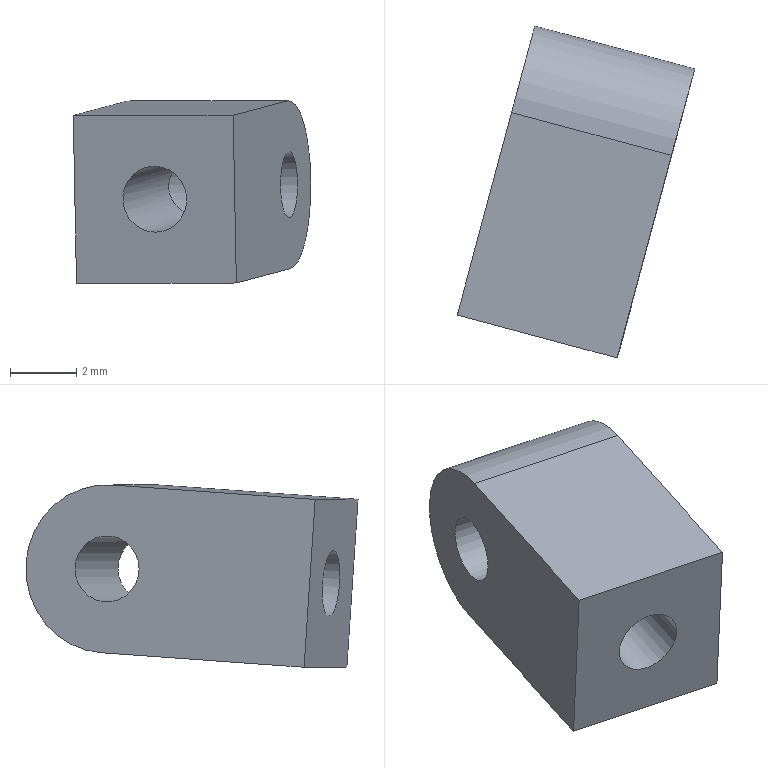Component | NX | BLOCK | 1 solid | 10 faces | box 7.18 x 10.03 x 5.52 mm | volume 179 mm3 | plane 5 | cylinder 3 | cone 2 | commonest cylinder face diameters 2 x2 5.08 x1
STEP:
#1=CARTESIAN_POINT('',(0.,0.,0.));
#2=DIRECTION('',(0.,0.,1.));
#3=DIRECTION('',(1.,0.,0.));
#4=AXIS2_PLACEMENT_3D('',#1,#2,#3);
#5=CARTESIAN_POINT('',(26.408,-132.214,153.506));
#6=VERTEX_POINT('',#5);
#7=CARTESIAN_POINT('',(28.048,-126.095,153.942));
#8=VERTEX_POINT('',#7);
#9=CARTESIAN_POINT('',(26.408,-132.214,153.506));
#10=DIRECTION('',(0.2582,0.9636,0.06876));
#11=VECTOR('',#10,1.);
#12=LINE('',#9,#11);
#13=CARTESIAN_POINT('',(21.579,-130.92,153.499));
#14=DIRECTION('',(0.01913,0.06606,-0.9976));
#15=DIRECTION('',(0.2582,0.9636,0.06876));
#16=AXIS2_PLACEMENT_3D('',#13,#14,#15);
#17=PLANE('',#16);
#18=CARTESIAN_POINT('',(0.,5.));
#19=DIRECTION('',(1.,0.));
#20=VECTOR('',#19,1.);
#21=LINE('',#18,#20);
#22=(GEOMETRIC_REPRESENTATION_CONTEXT(2)PARAMETRIC_REPRESENTATION_CONTEXT()REPRESENTATION_CONTEXT('',''));
#23=DEFINITIONAL_REPRESENTATION('',(#21),#22);
#24=PCURVE('',#17,#23);
#25=CARTESIAN_POINT('',(27.999,-126.263,156.476));
#26=DIRECTION('',(0.9659,-0.2589,0.001382));
#27=DIRECTION('',(0.2582,0.9636,0.06876));
#28=AXIS2_PLACEMENT_3D('',#25,#26,#27);
#29=PLANE('',#28);
#30=CARTESIAN_POINT('',(-6.35,-2.54));
#31=DIRECTION('',(1.,-0.));
#32=VECTOR('',#31,1.);
#33=LINE('',#30,#32);
#34=(GEOMETRIC_REPRESENTATION_CONTEXT(2)PARAMETRIC_REPRESENTATION_CONTEXT()REPRESENTATION_CONTEXT('',''));
#35=DEFINITIONAL_REPRESENTATION('',(#33),#34);
#36=PCURVE('',#29,#35);
#37=SURFACE_CURVE('',#12,(#24,#36),.PCURVE_S1.);
#38=EDGE_CURVE('',#6,#8,#37,.T.);
#39=ORIENTED_EDGE('',*,*,#38,.F.);
#40=CARTESIAN_POINT('',(21.579,-130.92,153.499));
#41=VERTEX_POINT('',#40);
#42=CARTESIAN_POINT('',(21.579,-130.92,153.499));
#43=DIRECTION('',(0.9659,-0.2589,0.001382));
#44=VECTOR('',#43,1.);
#45=LINE('',#42,#44);
#46=CARTESIAN_POINT('',(0.,0.));
#47=DIRECTION('',(-0.,1.));
#48=VECTOR('',#47,1.);
#49=LINE('',#46,#48);
#50=(GEOMETRIC_REPRESENTATION_CONTEXT(2)PARAMETRIC_REPRESENTATION_CONTEXT()REPRESENTATION_CONTEXT('',''));
#51=DEFINITIONAL_REPRESENTATION('',(#49),#50);
#52=PCURVE('',#17,#51);
#53=CARTESIAN_POINT('',(21.481,-131.255,158.567));
#54=DIRECTION('',(-0.2582,-0.9636,-0.06876));
#55=DIRECTION('',(0.01913,0.06606,-0.9976));
#56=AXIS2_PLACEMENT_3D('',#53,#54,#55);
#57=PLANE('',#56);
#58=CARTESIAN_POINT('',(5.08,0.));
#59=DIRECTION('',(-0.,1.));
#60=VECTOR('',#59,1.);
#61=LINE('',#58,#60);
#62=(GEOMETRIC_REPRESENTATION_CONTEXT(2)PARAMETRIC_REPRESENTATION_CONTEXT()REPRESENTATION_CONTEXT('',''));
#63=DEFINITIONAL_REPRESENTATION('',(#61),#62);
#64=PCURVE('',#57,#63);
#65=SURFACE_CURVE('',#45,(#52,#64),.PCURVE_S1.);
#66=EDGE_CURVE('',#41,#6,#65,.T.);
#67=ORIENTED_EDGE('',*,*,#66,.F.);
#68=CARTESIAN_POINT('',(23.218,-124.801,153.935));
#69=VERTEX_POINT('',#68);
#70=CARTESIAN_POINT('',(21.579,-130.92,153.499));
#71=DIRECTION('',(0.2582,0.9636,0.06876));
#72=VECTOR('',#71,1.);
#73=LINE('',#70,#72);
#74=CARTESIAN_POINT('',(0.,0.));
#75=DIRECTION('',(1.,0.));
#76=VECTOR('',#75,1.);
#77=LINE('',#74,#76);
#78=(GEOMETRIC_REPRESENTATION_CONTEXT(2)PARAMETRIC_REPRESENTATION_CONTEXT()REPRESENTATION_CONTEXT('',''));
#79=DEFINITIONAL_REPRESENTATION('',(#77),#78);
#80=PCURVE('',#17,#79);
#81=CARTESIAN_POINT('',(23.17,-124.969,156.469));
#82=DIRECTION('',(0.9659,-0.2589,0.001382));
#83=DIRECTION('',(0.2582,0.9636,0.06876));
#84=AXIS2_PLACEMENT_3D('',#81,#82,#83);
#85=PLANE('',#84);
#86=CARTESIAN_POINT('',(-6.35,-2.54));
#87=DIRECTION('',(1.,-0.));
#88=VECTOR('',#87,1.);
#89=LINE('',#86,#88);
#90=(GEOMETRIC_REPRESENTATION_CONTEXT(2)PARAMETRIC_REPRESENTATION_CONTEXT()REPRESENTATION_CONTEXT('',''));
#91=DEFINITIONAL_REPRESENTATION('',(#89),#90);
#92=PCURVE('',#85,#91);
#93=SURFACE_CURVE('',#73,(#80,#92),.PCURVE_S1.);
#94=EDGE_CURVE('',#41,#69,#93,.T.);
#95=ORIENTED_EDGE('',*,*,#94,.T.);
#96=CARTESIAN_POINT('',(23.218,-124.801,153.935));
#97=DIRECTION('',(0.9659,-0.2589,0.001382));
#98=VECTOR('',#97,1.);
#99=LINE('',#96,#98);
#100=CARTESIAN_POINT('',(6.35,-0.));
#101=DIRECTION('',(-0.,1.));
#102=VECTOR('',#101,1.);
#103=LINE('',#100,#102);
#104=(GEOMETRIC_REPRESENTATION_CONTEXT(2)PARAMETRIC_REPRESENTATION_CONTEXT()REPRESENTATION_CONTEXT('',''));
#105=DEFINITIONAL_REPRESENTATION('',(#103),#104);
#106=PCURVE('',#17,#105);
#107=CARTESIAN_POINT('',(23.17,-124.969,156.469));
#108=DIRECTION('',(0.9659,-0.2589,0.001382));
#109=DIRECTION('',(-0.01913,-0.06606,0.9976));
#110=AXIS2_PLACEMENT_3D('',#107,#108,#109);
#111=CYLINDRICAL_SURFACE('',#110,2.54);
#112=CARTESIAN_POINT('',(3.142,-0.));
#113=DIRECTION('',(-0.,1.));
#114=VECTOR('',#113,1.);
#115=LINE('',#112,#114);
#116=(GEOMETRIC_REPRESENTATION_CONTEXT(2)PARAMETRIC_REPRESENTATION_CONTEXT()REPRESENTATION_CONTEXT('',''));
#117=DEFINITIONAL_REPRESENTATION('',(#115),#116);
#118=PCURVE('',#111,#117);
#119=SURFACE_CURVE('',#99,(#106,#118),.PCURVE_S1.);
#120=EDGE_CURVE('',#69,#8,#119,.T.);
#121=ORIENTED_EDGE('',*,*,#120,.T.);
#122=EDGE_LOOP('',(#39,#67,#95,#121));
#123=FACE_BOUND('',#122,.T.);
#124=ADVANCED_FACE('',(#123),#17,.T.);
#125=CARTESIAN_POINT('',(27.951,-126.431,159.01));
#126=VERTEX_POINT('',#125);
#127=CARTESIAN_POINT('',(27.999,-126.263,156.476));
#128=DIRECTION('',(0.9659,-0.2589,0.001382));
#129=DIRECTION('',(0.2582,0.9636,0.06876));
#130=AXIS2_PLACEMENT_3D('',#127,#128,#129);
#131=CIRCLE('',#130,2.54);
#132=CARTESIAN_POINT('',(-1.571,5.));
#133=DIRECTION('',(1.,0.));
#134=VECTOR('',#133,1.);
#135=LINE('',#132,#134);
#136=(GEOMETRIC_REPRESENTATION_CONTEXT(2)PARAMETRIC_REPRESENTATION_CONTEXT()REPRESENTATION_CONTEXT('',''));
#137=DEFINITIONAL_REPRESENTATION('',(#135),#136);
#138=PCURVE('',#111,#137);
#139=CARTESIAN_POINT('',(0.,0.));
#140=DIRECTION('',(1.,0.));
#141=AXIS2_PLACEMENT_2D('',#139,#140);
#142=CIRCLE('',#141,2.54);
#143=(GEOMETRIC_REPRESENTATION_CONTEXT(2)PARAMETRIC_REPRESENTATION_CONTEXT()REPRESENTATION_CONTEXT('',''));
#144=DEFINITIONAL_REPRESENTATION('',(#142),#143);
#145=PCURVE('',#29,#144);
#146=SURFACE_CURVE('',#131,(#138,#145),.PCURVE_S1.);
#147=EDGE_CURVE('',#8,#126,#146,.T.);
#148=ORIENTED_EDGE('',*,*,#147,.F.);
#149=ORIENTED_EDGE('',*,*,#120,.F.);
#150=CARTESIAN_POINT('',(23.121,-125.136,159.003));
#151=VERTEX_POINT('',#150);
#152=CARTESIAN_POINT('',(23.17,-124.969,156.469));
#153=DIRECTION('',(0.9659,-0.2589,0.001382));
#154=DIRECTION('',(0.2582,0.9636,0.06876));
#155=AXIS2_PLACEMENT_3D('',#152,#153,#154);
#156=CIRCLE('',#155,2.54);
#157=CARTESIAN_POINT('',(-1.571,-0.));
#158=DIRECTION('',(1.,0.));
#159=VECTOR('',#158,1.);
#160=LINE('',#157,#159);
#161=(GEOMETRIC_REPRESENTATION_CONTEXT(2)PARAMETRIC_REPRESENTATION_CONTEXT()REPRESENTATION_CONTEXT('',''));
#162=DEFINITIONAL_REPRESENTATION('',(#160),#161);
#163=PCURVE('',#111,#162);
#164=CARTESIAN_POINT('',(0.,0.));
#165=DIRECTION('',(1.,0.));
#166=AXIS2_PLACEMENT_2D('',#164,#165);
#167=CIRCLE('',#166,2.54);
#168=(GEOMETRIC_REPRESENTATION_CONTEXT(2)PARAMETRIC_REPRESENTATION_CONTEXT()REPRESENTATION_CONTEXT('',''));
#169=DEFINITIONAL_REPRESENTATION('',(#167),#168);
#170=PCURVE('',#85,#169);
#171=SURFACE_CURVE('',#156,(#163,#170),.PCURVE_S1.);
#172=EDGE_CURVE('',#69,#151,#171,.T.);
#173=ORIENTED_EDGE('',*,*,#172,.T.);
#174=CARTESIAN_POINT('',(23.121,-125.136,159.003));
#175=DIRECTION('',(0.9659,-0.2589,0.001382));
#176=VECTOR('',#175,1.);
#177=LINE('',#174,#176);
#178=CARTESIAN_POINT('',(6.283,0.));
#179=DIRECTION('',(0.,1.));
#180=VECTOR('',#179,1.);
#181=LINE('',#178,#180);
#182=(GEOMETRIC_REPRESENTATION_CONTEXT(2)PARAMETRIC_REPRESENTATION_CONTEXT()REPRESENTATION_CONTEXT('',''));
#183=DEFINITIONAL_REPRESENTATION('',(#181),#182);
#184=PCURVE('',#111,#183);
#185=CARTESIAN_POINT('',(23.121,-125.136,159.003));
#186=DIRECTION('',(-0.01913,-0.06606,0.9976));
#187=DIRECTION('',(-0.2582,-0.9636,-0.06876));
#188=AXIS2_PLACEMENT_3D('',#185,#186,#187);
#189=PLANE('',#188);
#190=CARTESIAN_POINT('',(0.,0.));
#191=DIRECTION('',(0.,1.));
#192=VECTOR('',#191,1.);
#193=LINE('',#190,#192);
#194=(GEOMETRIC_REPRESENTATION_CONTEXT(2)PARAMETRIC_REPRESENTATION_CONTEXT()REPRESENTATION_CONTEXT('',''));
#195=DEFINITIONAL_REPRESENTATION('',(#193),#194);
#196=PCURVE('',#189,#195);
#197=SURFACE_CURVE('',#177,(#184,#196),.PCURVE_S1.);
#198=EDGE_CURVE('',#151,#126,#197,.T.);
#199=ORIENTED_EDGE('',*,*,#198,.T.);
#200=EDGE_LOOP('',(#148,#149,#173,#199));
#201=FACE_BOUND('',#200,.T.);
#202=ADVANCED_FACE('',(#201),#111,.T.);
#203=CARTESIAN_POINT('',(26.311,-132.55,158.574));
#204=VERTEX_POINT('',#203);
#205=CARTESIAN_POINT('',(27.951,-126.431,159.01));
#206=DIRECTION('',(-0.2582,-0.9636,-0.06876));
#207=VECTOR('',#206,1.);
#208=LINE('',#205,#207);
#209=CARTESIAN_POINT('',(-0.,5.));
#210=DIRECTION('',(1.,-0.));
#211=VECTOR('',#210,1.);
#212=LINE('',#209,#211);
#213=(GEOMETRIC_REPRESENTATION_CONTEXT(2)PARAMETRIC_REPRESENTATION_CONTEXT()REPRESENTATION_CONTEXT('',''));
#214=DEFINITIONAL_REPRESENTATION('',(#212),#213);
#215=PCURVE('',#189,#214);
#216=CARTESIAN_POINT('',(0.,2.54));
#217=DIRECTION('',(-1.,0.));
#218=VECTOR('',#217,1.);
#219=LINE('',#216,#218);
#220=(GEOMETRIC_REPRESENTATION_CONTEXT(2)PARAMETRIC_REPRESENTATION_CONTEXT()REPRESENTATION_CONTEXT('',''));
#221=DEFINITIONAL_REPRESENTATION('',(#219),#220);
#222=PCURVE('',#29,#221);
#223=SURFACE_CURVE('',#208,(#215,#222),.PCURVE_S1.);
#224=EDGE_CURVE('',#126,#204,#223,.T.);
#225=ORIENTED_EDGE('',*,*,#224,.F.);
#226=ORIENTED_EDGE('',*,*,#198,.F.);
#227=CARTESIAN_POINT('',(21.481,-131.255,158.567));
#228=VERTEX_POINT('',#227);
#229=CARTESIAN_POINT('',(23.121,-125.136,159.003));
#230=DIRECTION('',(-0.2582,-0.9636,-0.06876));
#231=VECTOR('',#230,1.);
#232=LINE('',#229,#231);
#233=CARTESIAN_POINT('',(0.,0.));
#234=DIRECTION('',(1.,-0.));
#235=VECTOR('',#234,1.);
#236=LINE('',#233,#235);
#237=(GEOMETRIC_REPRESENTATION_CONTEXT(2)PARAMETRIC_REPRESENTATION_CONTEXT()REPRESENTATION_CONTEXT('',''));
#238=DEFINITIONAL_REPRESENTATION('',(#236),#237);
#239=PCURVE('',#189,#238);
#240=CARTESIAN_POINT('',(0.,2.54));
#241=DIRECTION('',(-1.,0.));
#242=VECTOR('',#241,1.);
#243=LINE('',#240,#242);
#244=(GEOMETRIC_REPRESENTATION_CONTEXT(2)PARAMETRIC_REPRESENTATION_CONTEXT()REPRESENTATION_CONTEXT('',''));
#245=DEFINITIONAL_REPRESENTATION('',(#243),#244);
#246=PCURVE('',#85,#245);
#247=SURFACE_CURVE('',#232,(#239,#246),.PCURVE_S1.);
#248=EDGE_CURVE('',#151,#228,#247,.T.);
#249=ORIENTED_EDGE('',*,*,#248,.T.);
#250=CARTESIAN_POINT('',(21.481,-131.255,158.567));
#251=DIRECTION('',(0.9659,-0.2589,0.001382));
#252=VECTOR('',#251,1.);
#253=LINE('',#250,#252);
#254=CARTESIAN_POINT('',(6.35,-0.));
#255=DIRECTION('',(0.,1.));
#256=VECTOR('',#255,1.);
#257=LINE('',#254,#256);
#258=(GEOMETRIC_REPRESENTATION_CONTEXT(2)PARAMETRIC_REPRESENTATION_CONTEXT()REPRESENTATION_CONTEXT('',''));
#259=DEFINITIONAL_REPRESENTATION('',(#257),#258);
#260=PCURVE('',#189,#259);
#261=CARTESIAN_POINT('',(0.,0.));
#262=DIRECTION('',(-0.,1.));
#263=VECTOR('',#262,1.);
#264=LINE('',#261,#263);
#265=(GEOMETRIC_REPRESENTATION_CONTEXT(2)PARAMETRIC_REPRESENTATION_CONTEXT()REPRESENTATION_CONTEXT('',''));
#266=DEFINITIONAL_REPRESENTATION('',(#264),#265);
#267=PCURVE('',#57,#266);
#268=SURFACE_CURVE('',#253,(#260,#267),.PCURVE_S1.);
#269=EDGE_CURVE('',#228,#204,#268,.T.);
#270=ORIENTED_EDGE('',*,*,#269,.T.);
#271=EDGE_LOOP('',(#225,#226,#249,#270));
#272=FACE_BOUND('',#271,.T.);
#273=ADVANCED_FACE('',(#272),#189,.T.);
#274=CARTESIAN_POINT('',(23.926,-131.801,157.034));
#275=VERTEX_POINT('',#274);
#276=CARTESIAN_POINT('',(23.945,-131.735,156.036));
#277=DIRECTION('',(0.2582,0.9636,0.06876));
#278=DIRECTION('',(-0.01913,-0.06606,0.9976));
#279=AXIS2_PLACEMENT_3D('',#276,#277,#278);
#280=CIRCLE('',#279,1.);
#281=CARTESIAN_POINT('',(1.54,2.5));
#282=CARTESIAN_POINT('',(1.54,4.232));
#283=CARTESIAN_POINT('',(3.04,3.366));
#284=CARTESIAN_POINT('',(4.54,2.5));
#285=CARTESIAN_POINT('',(3.04,1.634));
#286=CARTESIAN_POINT('',(1.54,0.7679));
#287=CARTESIAN_POINT('',(1.54,2.5));
#288=(BOUNDED_CURVE()B_SPLINE_CURVE(2,(#281,#282,#283,#284,#285,#286,#287),.UNSPECIFIED.,.T.,.F.)B_SPLINE_CURVE_WITH_KNOTS((1,2,2,2,2,1),(-2.094,0.,2.094,4.189,6.283,8.378),.UNSPECIFIED.)CURVE()GEOMETRIC_REPRESENTATION_ITEM()RATIONAL_B_SPLINE_CURVE((1.,0.5,1.,0.5,1.,0.5,1.))REPRESENTATION_ITEM(''));
#289=(GEOMETRIC_REPRESENTATION_CONTEXT(2)PARAMETRIC_REPRESENTATION_CONTEXT()REPRESENTATION_CONTEXT('',''));
#290=DEFINITIONAL_REPRESENTATION('',(#288),#289);
#291=PCURVE('',#57,#290);
#292=CARTESIAN_POINT('',(23.945,-131.735,156.036));
#293=DIRECTION('',(0.2582,0.9636,0.06876));
#294=DIRECTION('',(-0.01913,-0.06606,0.9976));
#295=AXIS2_PLACEMENT_3D('',#292,#293,#294);
#296=CYLINDRICAL_SURFACE('',#295,1.);
#297=CARTESIAN_POINT('',(0.,0.));
#298=DIRECTION('',(1.,0.));
#299=VECTOR('',#298,1.);
#300=LINE('',#297,#299);
#301=(GEOMETRIC_REPRESENTATION_CONTEXT(2)PARAMETRIC_REPRESENTATION_CONTEXT()REPRESENTATION_CONTEXT('',''));
#302=DEFINITIONAL_REPRESENTATION('',(#300),#301);
#303=PCURVE('',#296,#302);
#304=SURFACE_CURVE('',#280,(#291,#303),.PCURVE_S1.);
#305=EDGE_CURVE('',#275,#275,#304,.T.);
#306=ORIENTED_EDGE('',*,*,#305,.T.);
#307=EDGE_LOOP('',(#306));
#308=FACE_BOUND('',#307,.T.);
#309=CARTESIAN_POINT('',(26.311,-132.55,158.574));
#310=DIRECTION('',(0.01913,0.06606,-0.9976));
#311=VECTOR('',#310,1.);
#312=LINE('',#309,#311);
#313=CARTESIAN_POINT('',(-0.,5.));
#314=DIRECTION('',(1.,-0.));
#315=VECTOR('',#314,1.);
#316=LINE('',#313,#315);
#317=(GEOMETRIC_REPRESENTATION_CONTEXT(2)PARAMETRIC_REPRESENTATION_CONTEXT()REPRESENTATION_CONTEXT('',''));
#318=DEFINITIONAL_REPRESENTATION('',(#316),#317);
#319=PCURVE('',#57,#318);
#320=CARTESIAN_POINT('',(-6.35,2.54));
#321=DIRECTION('',(0.,-1.));
#322=VECTOR('',#321,1.);
#323=LINE('',#320,#322);
#324=(GEOMETRIC_REPRESENTATION_CONTEXT(2)PARAMETRIC_REPRESENTATION_CONTEXT()REPRESENTATION_CONTEXT('',''));
#325=DEFINITIONAL_REPRESENTATION('',(#323),#324);
#326=PCURVE('',#29,#325);
#327=SURFACE_CURVE('',#312,(#319,#326),.PCURVE_S1.);
#328=EDGE_CURVE('',#204,#6,#327,.T.);
#329=ORIENTED_EDGE('',*,*,#328,.F.);
#330=ORIENTED_EDGE('',*,*,#269,.F.);
#331=CARTESIAN_POINT('',(21.481,-131.255,158.567));
#332=DIRECTION('',(0.01913,0.06606,-0.9976));
#333=VECTOR('',#332,1.);
#334=LINE('',#331,#333);
#335=CARTESIAN_POINT('',(0.,0.));
#336=DIRECTION('',(1.,-0.));
#337=VECTOR('',#336,1.);
#338=LINE('',#335,#337);
#339=(GEOMETRIC_REPRESENTATION_CONTEXT(2)PARAMETRIC_REPRESENTATION_CONTEXT()REPRESENTATION_CONTEXT('',''));
#340=DEFINITIONAL_REPRESENTATION('',(#338),#339);
#341=PCURVE('',#57,#340);
#342=CARTESIAN_POINT('',(-6.35,2.54));
#343=DIRECTION('',(0.,-1.));
#344=VECTOR('',#343,1.);
#345=LINE('',#342,#344);
#346=(GEOMETRIC_REPRESENTATION_CONTEXT(2)PARAMETRIC_REPRESENTATION_CONTEXT()REPRESENTATION_CONTEXT('',''));
#347=DEFINITIONAL_REPRESENTATION('',(#345),#346);
#348=PCURVE('',#85,#347);
#349=SURFACE_CURVE('',#334,(#341,#348),.PCURVE_S1.);
#350=EDGE_CURVE('',#228,#41,#349,.T.);
#351=ORIENTED_EDGE('',*,*,#350,.T.);
#352=ORIENTED_EDGE('',*,*,#66,.T.);
#353=EDGE_LOOP('',(#329,#330,#351,#352));
#354=FACE_BOUND('',#353,.T.);
#355=ADVANCED_FACE('',(#308,#354),#57,.T.);
#356=CARTESIAN_POINT('',(23.429,-124.003,156.469));
#357=VERTEX_POINT('',#356);
#358=CARTESIAN_POINT('',(23.17,-124.969,156.469));
#359=DIRECTION('',(0.9659,-0.2589,0.001382));
#360=DIRECTION('',(0.2589,0.9659,0.00000007));
#361=AXIS2_PLACEMENT_3D('',#358,#359,#360);
#362=CIRCLE('',#361,1.);
#363=CARTESIAN_POINT('',(23.17,-124.969,156.469));
#364=DIRECTION('',(0.9659,-0.2589,0.001382));
#365=DIRECTION('',(-0.01913,-0.06606,0.9976));
#366=AXIS2_PLACEMENT_3D('',#363,#364,#365);
#367=CYLINDRICAL_SURFACE('',#366,1.);
#368=CARTESIAN_POINT('',(4.644,0.));
#369=DIRECTION('',(1.,0.));
#370=VECTOR('',#369,1.);
#371=LINE('',#368,#370);
#372=(GEOMETRIC_REPRESENTATION_CONTEXT(2)PARAMETRIC_REPRESENTATION_CONTEXT()REPRESENTATION_CONTEXT('',''));
#373=DEFINITIONAL_REPRESENTATION('',(#371),#372);
#374=PCURVE('',#367,#373);
#375=CARTESIAN_POINT('',(0.,-0.));
#376=DIRECTION('',(0.9976,-0.06876));
#377=AXIS2_PLACEMENT_2D('',#375,#376);
#378=CIRCLE('',#377,1.);
#379=(GEOMETRIC_REPRESENTATION_CONTEXT(2)PARAMETRIC_REPRESENTATION_CONTEXT()REPRESENTATION_CONTEXT('',''));
#380=DEFINITIONAL_REPRESENTATION('',(#378),#379);
#381=PCURVE('',#85,#380);
#382=SURFACE_CURVE('',#362,(#374,#381),.PCURVE_S1.);
#383=EDGE_CURVE('',#357,#357,#382,.T.);
#384=ORIENTED_EDGE('',*,*,#383,.T.);
#385=CARTESIAN_POINT('',(28.258,-125.297,156.476));
#386=VERTEX_POINT('',#385);
#387=CARTESIAN_POINT('',(23.429,-124.003,156.469));
#388=CARTESIAN_POINT('',(28.258,-125.297,156.476));
#389=B_SPLINE_CURVE_WITH_KNOTS('',1,(#387,#388),.UNSPECIFIED.,.F.,.F.,(2,2),(0.,5.),.PIECEWISE_BEZIER_KNOTS.);
#390=CARTESIAN_POINT('',(10.927,0.));
#391=DIRECTION('',(0.,1.));
#392=VECTOR('',#391,1.);
#393=LINE('',#390,#392);
#394=(GEOMETRIC_REPRESENTATION_CONTEXT(2)PARAMETRIC_REPRESENTATION_CONTEXT()REPRESENTATION_CONTEXT('',''));
#395=DEFINITIONAL_REPRESENTATION('',(#393),#394);
#396=PCURVE('',#367,#395);
#397=CARTESIAN_POINT('',(4.644,0.));
#398=DIRECTION('',(0.,1.));
#399=VECTOR('',#398,1.);
#400=LINE('',#397,#399);
#401=(GEOMETRIC_REPRESENTATION_CONTEXT(2)PARAMETRIC_REPRESENTATION_CONTEXT()REPRESENTATION_CONTEXT('',''));
#402=DEFINITIONAL_REPRESENTATION('',(#400),#401);
#403=PCURVE('',#367,#402);
#404=SEAM_CURVE('',#389,(#396,#403),.PCURVE_S1.);
#405=EDGE_CURVE('',#357,#386,#404,.T.);
#406=ORIENTED_EDGE('',*,*,#405,.T.);
#407=CARTESIAN_POINT('',(27.999,-126.263,156.476));
#408=DIRECTION('',(0.9659,-0.2589,0.001382));
#409=DIRECTION('',(0.2589,0.9659,0.00000007));
#410=AXIS2_PLACEMENT_3D('',#407,#408,#409);
#411=CIRCLE('',#410,1.);
#412=CARTESIAN_POINT('',(4.644,5.));
#413=DIRECTION('',(1.,0.));
#414=VECTOR('',#413,1.);
#415=LINE('',#412,#414);
#416=(GEOMETRIC_REPRESENTATION_CONTEXT(2)PARAMETRIC_REPRESENTATION_CONTEXT()REPRESENTATION_CONTEXT('',''));
#417=DEFINITIONAL_REPRESENTATION('',(#415),#416);
#418=PCURVE('',#367,#417);
#419=CARTESIAN_POINT('',(0.,-0.));
#420=DIRECTION('',(0.9976,-0.06876));
#421=AXIS2_PLACEMENT_2D('',#419,#420);
#422=CIRCLE('',#421,1.);
#423=(GEOMETRIC_REPRESENTATION_CONTEXT(2)PARAMETRIC_REPRESENTATION_CONTEXT()REPRESENTATION_CONTEXT('',''));
#424=DEFINITIONAL_REPRESENTATION('',(#422),#423);
#425=PCURVE('',#29,#424);
#426=SURFACE_CURVE('',#411,(#418,#425),.PCURVE_S1.);
#427=EDGE_CURVE('',#386,#386,#426,.T.);
#428=ORIENTED_EDGE('',*,*,#427,.F.);
#429=ORIENTED_EDGE('',*,*,#405,.F.);
#430=EDGE_LOOP('',(#384,#406,#428,#429));
#431=FACE_BOUND('',#430,.F.);
#432=CARTESIAN_POINT('',(25.138,-125.924,157.383));
#433=VERTEX_POINT('',#432);
#434=CARTESIAN_POINT('',(25.174,-125.801,155.514));
#435=VERTEX_POINT('',#434);
#436=CARTESIAN_POINT('',(25.584,-125.616,156.473));
#437=DIRECTION('',(0.5004,-0.8645,-0.04764));
#438=DIRECTION('',(0.8656,0.4983,0.0496));
#439=AXIS2_PLACEMENT_3D('',#436,#437,#438);
#440=ELLIPSE('',#439,1.414,1.);
#441=CARTESIAN_POINT('',(6.641,2.15));
#442=CARTESIAN_POINT('',(6.678,2.116));
#443=CARTESIAN_POINT('',(6.751,2.048));
#444=CARTESIAN_POINT('',(6.861,1.952));
#445=CARTESIAN_POINT('',(6.972,1.863));
#446=CARTESIAN_POINT('',(7.082,1.782));
#447=CARTESIAN_POINT('',(7.192,1.709));
#448=CARTESIAN_POINT('',(7.303,1.647));
#449=CARTESIAN_POINT('',(7.413,1.594));
#450=CARTESIAN_POINT('',(7.523,1.552));
#451=CARTESIAN_POINT('',(7.633,1.522));
#452=CARTESIAN_POINT('',(7.744,1.504));
#453=CARTESIAN_POINT('',(7.854,1.498));
#454=CARTESIAN_POINT('',(7.964,1.504));
#455=CARTESIAN_POINT('',(8.075,1.522));
#456=CARTESIAN_POINT('',(8.185,1.552));
#457=CARTESIAN_POINT('',(8.295,1.594));
#458=CARTESIAN_POINT('',(8.405,1.647));
#459=CARTESIAN_POINT('',(8.516,1.709));
#460=CARTESIAN_POINT('',(8.626,1.782));
#461=CARTESIAN_POINT('',(8.736,1.863));
#462=CARTESIAN_POINT('',(8.847,1.952));
#463=CARTESIAN_POINT('',(8.957,2.048));
#464=CARTESIAN_POINT('',(9.03,2.116));
#465=CARTESIAN_POINT('',(9.067,2.15));
#466=B_SPLINE_CURVE_WITH_KNOTS('',3,(#441,#442,#443,#444,#445,#446,#447,#448,#449,#450,#451,#452,#453,#454,#455,#456,#457,#458,#459,#460,#461,#462,#463,#464,#465),.UNSPECIFIED.,.F.,.F.,(4,1,1,1,1,1,1,1,1,1,1,1,1,1,1,1,1,1,1,1,1,1,4),(1.928,2.039,2.149,2.259,2.37,2.48,2.59,2.7,2.811,2.921,3.031,3.142,3.252,3.362,3.472,3.583,3.693,3.803,3.914,4.024,4.134,4.245,4.355),.QUASI_UNIFORM_KNOTS.);
#467=(GEOMETRIC_REPRESENTATION_CONTEXT(2)PARAMETRIC_REPRESENTATION_CONTEXT()REPRESENTATION_CONTEXT('',''));
#468=DEFINITIONAL_REPRESENTATION('',(#466),#467);
#469=PCURVE('',#367,#468);
#470=CARTESIAN_POINT('',(5.926,6.));
#471=CARTESIAN_POINT('',(5.889,5.966));
#472=CARTESIAN_POINT('',(5.815,5.898));
#473=CARTESIAN_POINT('',(5.705,5.802));
#474=CARTESIAN_POINT('',(5.595,5.713));
#475=CARTESIAN_POINT('',(5.484,5.632));
#476=CARTESIAN_POINT('',(5.374,5.559));
#477=CARTESIAN_POINT('',(5.264,5.497));
#478=CARTESIAN_POINT('',(5.154,5.444));
#479=CARTESIAN_POINT('',(5.043,5.402));
#480=CARTESIAN_POINT('',(4.933,5.372));
#481=CARTESIAN_POINT('',(4.823,5.354));
#482=CARTESIAN_POINT('',(4.712,5.348));
#483=CARTESIAN_POINT('',(4.602,5.354));
#484=CARTESIAN_POINT('',(4.492,5.372));
#485=CARTESIAN_POINT('',(4.382,5.402));
#486=CARTESIAN_POINT('',(4.271,5.444));
#487=CARTESIAN_POINT('',(4.161,5.497));
#488=CARTESIAN_POINT('',(4.051,5.559));
#489=CARTESIAN_POINT('',(3.94,5.632));
#490=CARTESIAN_POINT('',(3.83,5.713));
#491=CARTESIAN_POINT('',(3.72,5.802));
#492=CARTESIAN_POINT('',(3.609,5.898));
#493=CARTESIAN_POINT('',(3.536,5.966));
#494=CARTESIAN_POINT('',(3.499,6.));
#495=B_SPLINE_CURVE_WITH_KNOTS('',3,(#470,#471,#472,#473,#474,#475,#476,#477,#478,#479,#480,#481,#482,#483,#484,#485,#486,#487,#488,#489,#490,#491,#492,#493,#494),.UNSPECIFIED.,.F.,.F.,(4,1,1,1,1,1,1,1,1,1,1,1,1,1,1,1,1,1,1,1,1,1,4),(1.928,2.039,2.149,2.259,2.37,2.48,2.59,2.7,2.811,2.921,3.031,3.142,3.252,3.362,3.472,3.583,3.693,3.803,3.914,4.024,4.134,4.245,4.355),.QUASI_UNIFORM_KNOTS.);
#496=(GEOMETRIC_REPRESENTATION_CONTEXT(2)PARAMETRIC_REPRESENTATION_CONTEXT()REPRESENTATION_CONTEXT('',''));
#497=DEFINITIONAL_REPRESENTATION('',(#495),#496);
#498=PCURVE('',#296,#497);
#499=SURFACE_CURVE('',#440,(#469,#498),.PCURVE_S1.);
#500=EDGE_CURVE('',#433,#435,#499,.T.);
#501=ORIENTED_EDGE('',*,*,#500,.F.);
#502=CARTESIAN_POINT('',(25.814,-126.106,157.384));
#503=VERTEX_POINT('',#502);
#504=CARTESIAN_POINT('',(25.814,-126.106,157.384));
#505=CARTESIAN_POINT('',(25.716,-126.061,157.392));
#506=CARTESIAN_POINT('',(25.614,-126.022,157.396));
#507=CARTESIAN_POINT('',(25.509,-125.993,157.396));
#508=CARTESIAN_POINT('',(25.388,-125.958,157.397));
#509=CARTESIAN_POINT('',(25.263,-125.936,157.392));
#510=CARTESIAN_POINT('',(25.138,-125.924,157.383));
#511=B_SPLINE_CURVE_WITH_KNOTS('',3,(#504,#505,#506,#507,#508,#509,#510),.UNSPECIFIED.,.F.,.F.,(4,3,4),(0.,0.4619,1.),.UNSPECIFIED.);
#512=CARTESIAN_POINT('',(6.641,2.85));
#513=CARTESIAN_POINT('',(6.639,2.84));
#514=CARTESIAN_POINT('',(6.635,2.818));
#515=CARTESIAN_POINT('',(6.63,2.787));
#516=CARTESIAN_POINT('',(6.625,2.755));
#517=CARTESIAN_POINT('',(6.621,2.723));
#518=CARTESIAN_POINT('',(6.618,2.692));
#519=CARTESIAN_POINT('',(6.615,2.66));
#520=CARTESIAN_POINT('',(6.612,2.628));
#521=CARTESIAN_POINT('',(6.61,2.596));
#522=CARTESIAN_POINT('',(6.609,2.564));
#523=CARTESIAN_POINT('',(6.608,2.532));
#524=CARTESIAN_POINT('',(6.607,2.5));
#525=CARTESIAN_POINT('',(6.608,2.468));
#526=CARTESIAN_POINT('',(6.609,2.436));
#527=CARTESIAN_POINT('',(6.61,2.404));
#528=CARTESIAN_POINT('',(6.612,2.372));
#529=CARTESIAN_POINT('',(6.615,2.34));
#530=CARTESIAN_POINT('',(6.618,2.308));
#531=CARTESIAN_POINT('',(6.621,2.276));
#532=CARTESIAN_POINT('',(6.625,2.245));
#533=CARTESIAN_POINT('',(6.63,2.213));
#534=CARTESIAN_POINT('',(6.635,2.181));
#535=CARTESIAN_POINT('',(6.639,2.16));
#536=CARTESIAN_POINT('',(6.641,2.15));
#537=B_SPLINE_CURVE_WITH_KNOTS('',3,(#512,#513,#514,#515,#516,#517,#518,#519,#520,#521,#522,#523,#524,#525,#526,#527,#528,#529,#530,#531,#532,#533,#534,#535,#536),.UNSPECIFIED.,.F.,.F.,(4,1,1,1,1,1,1,1,1,1,1,1,1,1,1,1,1,1,1,1,1,1,4),(0.,0.04545,0.09091,0.1364,0.1818,0.2273,0.2727,0.3182,0.3636,0.4091,0.4545,0.5,0.5455,0.5909,0.6364,0.6818,0.7273,0.7727,0.8182,0.8636,0.9091,0.9545,1.),.QUASI_UNIFORM_KNOTS.);
#538=(GEOMETRIC_REPRESENTATION_CONTEXT(2)PARAMETRIC_REPRESENTATION_CONTEXT()REPRESENTATION_CONTEXT('',''));
#539=DEFINITIONAL_REPRESENTATION('',(#537),#538);
#540=PCURVE('',#367,#539);
#541=CARTESIAN_POINT('',(25.494,-125.953,156.449));
#542=DIRECTION('',(-0.2582,-0.9636,-0.06876));
#543=DIRECTION('',(0.01913,0.06606,-0.9976));
#544=AXIS2_PLACEMENT_3D('',#541,#542,#543);
#545=CONICAL_SURFACE('',#544,1.,1.03);
#546=CARTESIAN_POINT('',(2.784,-0.));
#547=CARTESIAN_POINT('',(2.794,-0.001823));
#548=CARTESIAN_POINT('',(2.814,-0.005328));
#549=CARTESIAN_POINT('',(2.845,-0.01015));
#550=CARTESIAN_POINT('',(2.877,-0.01451));
#551=CARTESIAN_POINT('',(2.909,-0.01841));
#552=CARTESIAN_POINT('',(2.942,-0.02182));
#553=CARTESIAN_POINT('',(2.974,-0.02473));
#554=CARTESIAN_POINT('',(3.008,-0.02712));
#555=CARTESIAN_POINT('',(3.041,-0.029));
#556=CARTESIAN_POINT('',(3.074,-0.03035));
#557=CARTESIAN_POINT('',(3.108,-0.03115));
#558=CARTESIAN_POINT('',(3.142,-0.03141));
#559=CARTESIAN_POINT('',(3.176,-0.03113));
#560=CARTESIAN_POINT('',(3.209,-0.03031));
#561=CARTESIAN_POINT('',(3.243,-0.02896));
#562=CARTESIAN_POINT('',(3.276,-0.02708));
#563=CARTESIAN_POINT('',(3.309,-0.02468));
#564=CARTESIAN_POINT('',(3.342,-0.02177));
#565=CARTESIAN_POINT('',(3.374,-0.01837));
#566=CARTESIAN_POINT('',(3.406,-0.01448));
#567=CARTESIAN_POINT('',(3.438,-0.01012));
#568=CARTESIAN_POINT('',(3.469,-0.005314));
#569=CARTESIAN_POINT('',(3.489,-0.001818));
#570=CARTESIAN_POINT('',(3.499,-0.));
#571=B_SPLINE_CURVE_WITH_KNOTS('',3,(#546,#547,#548,#549,#550,#551,#552,#553,#554,#555,#556,#557,#558,#559,#560,#561,#562,#563,#564,#565,#566,#567,#568,#569,#570),.UNSPECIFIED.,.F.,.F.,(4,1,1,1,1,1,1,1,1,1,1,1,1,1,1,1,1,1,1,1,1,1,4),(0.,0.04545,0.09091,0.1364,0.1818,0.2273,0.2727,0.3182,0.3636,0.4091,0.4545,0.5,0.5455,0.5909,0.6364,0.6818,0.7273,0.7727,0.8182,0.8636,0.9091,0.9545,1.),.QUASI_UNIFORM_KNOTS.);
#572=(GEOMETRIC_REPRESENTATION_CONTEXT(2)PARAMETRIC_REPRESENTATION_CONTEXT()REPRESENTATION_CONTEXT('',''));
#573=DEFINITIONAL_REPRESENTATION('',(#571),#572);
#574=PCURVE('',#545,#573);
#575=SURFACE_CURVE('',#511,(#540,#574),.PCURVE_S1.);
#576=EDGE_CURVE('',#503,#433,#575,.T.);
#577=ORIENTED_EDGE('',*,*,#576,.F.);
#578=CARTESIAN_POINT('',(25.85,-125.982,155.515));
#579=VERTEX_POINT('',#578);
#580=CARTESIAN_POINT('',(25.584,-125.616,156.473));
#581=DIRECTION('',(-0.8656,-0.4983,-0.0496));
#582=DIRECTION('',(0.5004,-0.8645,-0.04764));
#583=AXIS2_PLACEMENT_3D('',#580,#581,#582);
#584=ELLIPSE('',#583,1.414,1.);
#585=CARTESIAN_POINT('',(9.067,2.85));
#586=CARTESIAN_POINT('',(9.03,2.884));
#587=CARTESIAN_POINT('',(8.957,2.952));
#588=CARTESIAN_POINT('',(8.847,3.048));
#589=CARTESIAN_POINT('',(8.736,3.137));
#590=CARTESIAN_POINT('',(8.626,3.218));
#591=CARTESIAN_POINT('',(8.516,3.291));
#592=CARTESIAN_POINT('',(8.405,3.353));
#593=CARTESIAN_POINT('',(8.295,3.406));
#594=CARTESIAN_POINT('',(8.185,3.448));
#595=CARTESIAN_POINT('',(8.075,3.478));
#596=CARTESIAN_POINT('',(7.964,3.496));
#597=CARTESIAN_POINT('',(7.854,3.502));
#598=CARTESIAN_POINT('',(7.744,3.496));
#599=CARTESIAN_POINT('',(7.633,3.478));
#600=CARTESIAN_POINT('',(7.523,3.448));
#601=CARTESIAN_POINT('',(7.413,3.406));
#602=CARTESIAN_POINT('',(7.303,3.353));
#603=CARTESIAN_POINT('',(7.192,3.291));
#604=CARTESIAN_POINT('',(7.082,3.218));
#605=CARTESIAN_POINT('',(6.972,3.137));
#606=CARTESIAN_POINT('',(6.861,3.048));
#607=CARTESIAN_POINT('',(6.751,2.952));
#608=CARTESIAN_POINT('',(6.678,2.884));
#609=CARTESIAN_POINT('',(6.641,2.85));
#610=B_SPLINE_CURVE_WITH_KNOTS('',3,(#585,#586,#587,#588,#589,#590,#591,#592,#593,#594,#595,#596,#597,#598,#599,#600,#601,#602,#603,#604,#605,#606,#607,#608,#609),.UNSPECIFIED.,.F.,.F.,(4,1,1,1,1,1,1,1,1,1,1,1,1,1,1,1,1,1,1,1,1,1,4),(5.07,5.18,5.291,5.401,5.511,5.621,5.732,5.842,5.952,6.063,6.173,6.283,6.393,6.504,6.614,6.724,6.835,6.945,7.055,7.166,7.276,7.386,7.496),.QUASI_UNIFORM_KNOTS.);
#611=(GEOMETRIC_REPRESENTATION_CONTEXT(2)PARAMETRIC_REPRESENTATION_CONTEXT()REPRESENTATION_CONTEXT('',''));
#612=DEFINITIONAL_REPRESENTATION('',(#610),#611);
#613=PCURVE('',#367,#612);
#614=CARTESIAN_POINT('',(2.784,6.));
#615=CARTESIAN_POINT('',(2.747,5.966));
#616=CARTESIAN_POINT('',(2.674,5.898));
#617=CARTESIAN_POINT('',(2.563,5.802));
#618=CARTESIAN_POINT('',(2.453,5.713));
#619=CARTESIAN_POINT('',(2.343,5.632));
#620=CARTESIAN_POINT('',(2.233,5.559));
#621=CARTESIAN_POINT('',(2.122,5.497));
#622=CARTESIAN_POINT('',(2.012,5.444));
#623=CARTESIAN_POINT('',(1.902,5.402));
#624=CARTESIAN_POINT('',(1.791,5.372));
#625=CARTESIAN_POINT('',(1.681,5.354));
#626=CARTESIAN_POINT('',(1.571,5.348));
#627=CARTESIAN_POINT('',(1.461,5.354));
#628=CARTESIAN_POINT('',(1.35,5.372));
#629=CARTESIAN_POINT('',(1.24,5.402));
#630=CARTESIAN_POINT('',(1.13,5.444));
#631=CARTESIAN_POINT('',(1.019,5.497));
#632=CARTESIAN_POINT('',(0.909,5.559));
#633=CARTESIAN_POINT('',(0.7987,5.632));
#634=CARTESIAN_POINT('',(0.6885,5.713));
#635=CARTESIAN_POINT('',(0.5782,5.802));
#636=CARTESIAN_POINT('',(0.4679,5.898));
#637=CARTESIAN_POINT('',(0.3943,5.966));
#638=CARTESIAN_POINT('',(0.3576,6.));
#639=B_SPLINE_CURVE_WITH_KNOTS('',3,(#614,#615,#616,#617,#618,#619,#620,#621,#622,#623,#624,#625,#626,#627,#628,#629,#630,#631,#632,#633,#634,#635,#636,#637,#638),.UNSPECIFIED.,.F.,.F.,(4,1,1,1,1,1,1,1,1,1,1,1,1,1,1,1,1,1,1,1,1,1,4),(5.07,5.18,5.291,5.401,5.511,5.621,5.732,5.842,5.952,6.063,6.173,6.283,6.393,6.504,6.614,6.724,6.835,6.945,7.055,7.166,7.276,7.386,7.496),.QUASI_UNIFORM_KNOTS.);
#640=(GEOMETRIC_REPRESENTATION_CONTEXT(2)PARAMETRIC_REPRESENTATION_CONTEXT()REPRESENTATION_CONTEXT('',''));
#641=DEFINITIONAL_REPRESENTATION('',(#639),#640);
#642=PCURVE('',#296,#641);
#643=SURFACE_CURVE('',#584,(#613,#642),.PCURVE_S1.);
#644=EDGE_CURVE('',#579,#503,#643,.T.);
#645=ORIENTED_EDGE('',*,*,#644,.F.);
#646=CARTESIAN_POINT('',(25.174,-125.801,155.514));
#647=CARTESIAN_POINT('',(25.282,-125.81,155.508));
#648=CARTESIAN_POINT('',(25.39,-125.827,155.506));
#649=CARTESIAN_POINT('',(25.495,-125.854,155.505));
#650=CARTESIAN_POINT('',(25.617,-125.885,155.505));
#651=CARTESIAN_POINT('',(25.736,-125.929,155.508));
#652=CARTESIAN_POINT('',(25.85,-125.982,155.515));
#653=B_SPLINE_CURVE_WITH_KNOTS('',3,(#646,#647,#648,#649,#650,#651,#652),.UNSPECIFIED.,.F.,.F.,(4,3,4),(0.,0.4619,1.),.UNSPECIFIED.);
#654=CARTESIAN_POINT('',(9.067,2.15));
#655=CARTESIAN_POINT('',(9.069,2.16));
#656=CARTESIAN_POINT('',(9.073,2.182));
#657=CARTESIAN_POINT('',(9.078,2.213));
#658=CARTESIAN_POINT('',(9.083,2.245));
#659=CARTESIAN_POINT('',(9.087,2.277));
#660=CARTESIAN_POINT('',(9.09,2.308));
#661=CARTESIAN_POINT('',(9.093,2.34));
#662=CARTESIAN_POINT('',(9.096,2.372));
#663=CARTESIAN_POINT('',(9.098,2.404));
#664=CARTESIAN_POINT('',(9.099,2.436));
#665=CARTESIAN_POINT('',(9.1,2.468));
#666=CARTESIAN_POINT('',(9.101,2.5));
#667=CARTESIAN_POINT('',(9.1,2.532));
#668=CARTESIAN_POINT('',(9.099,2.564));
#669=CARTESIAN_POINT('',(9.098,2.596));
#670=CARTESIAN_POINT('',(9.096,2.628));
#671=CARTESIAN_POINT('',(9.093,2.66));
#672=CARTESIAN_POINT('',(9.09,2.692));
#673=CARTESIAN_POINT('',(9.087,2.724));
#674=CARTESIAN_POINT('',(9.083,2.755));
#675=CARTESIAN_POINT('',(9.078,2.787));
#676=CARTESIAN_POINT('',(9.073,2.819));
#677=CARTESIAN_POINT('',(9.069,2.84));
#678=CARTESIAN_POINT('',(9.067,2.85));
#679=B_SPLINE_CURVE_WITH_KNOTS('',3,(#654,#655,#656,#657,#658,#659,#660,#661,#662,#663,#664,#665,#666,#667,#668,#669,#670,#671,#672,#673,#674,#675,#676,#677,#678),.UNSPECIFIED.,.F.,.F.,(4,1,1,1,1,1,1,1,1,1,1,1,1,1,1,1,1,1,1,1,1,1,4),(0.,0.04545,0.09091,0.1364,0.1818,0.2273,0.2727,0.3182,0.3636,0.4091,0.4545,0.5,0.5455,0.5909,0.6364,0.6818,0.7273,0.7727,0.8182,0.8636,0.9091,0.9545,1.),.QUASI_UNIFORM_KNOTS.);
#680=(GEOMETRIC_REPRESENTATION_CONTEXT(2)PARAMETRIC_REPRESENTATION_CONTEXT()REPRESENTATION_CONTEXT('',''));
#681=DEFINITIONAL_REPRESENTATION('',(#679),#680);
#682=PCURVE('',#367,#681);
#683=CARTESIAN_POINT('',(25.494,-125.953,156.449));
#684=DIRECTION('',(-0.2582,-0.9636,-0.06876));
#685=DIRECTION('',(0.01913,0.06606,-0.9976));
#686=AXIS2_PLACEMENT_3D('',#683,#684,#685);
#687=CONICAL_SURFACE('',#686,1.,1.03);
#688=CARTESIAN_POINT('',(5.926,-0.));
#689=CARTESIAN_POINT('',(5.936,-0.001823));
#690=CARTESIAN_POINT('',(5.956,-0.005328));
#691=CARTESIAN_POINT('',(5.987,-0.01015));
#692=CARTESIAN_POINT('',(6.019,-0.01451));
#693=CARTESIAN_POINT('',(6.051,-0.01841));
#694=CARTESIAN_POINT('',(6.083,-0.02182));
#695=CARTESIAN_POINT('',(6.116,-0.02473));
#696=CARTESIAN_POINT('',(6.149,-0.02712));
#697=CARTESIAN_POINT('',(6.183,-0.029));
#698=CARTESIAN_POINT('',(6.216,-0.03035));
#699=CARTESIAN_POINT('',(6.25,-0.03115));
#700=CARTESIAN_POINT('',(6.283,-0.03141));
#701=CARTESIAN_POINT('',(6.317,-0.03113));
#702=CARTESIAN_POINT('',(6.351,-0.03031));
#703=CARTESIAN_POINT('',(6.384,-0.02896));
#704=CARTESIAN_POINT('',(6.418,-0.02708));
#705=CARTESIAN_POINT('',(6.451,-0.02468));
#706=CARTESIAN_POINT('',(6.484,-0.02177));
#707=CARTESIAN_POINT('',(6.516,-0.01837));
#708=CARTESIAN_POINT('',(6.548,-0.01448));
#709=CARTESIAN_POINT('',(6.579,-0.01012));
#710=CARTESIAN_POINT('',(6.61,-0.005314));
#711=CARTESIAN_POINT('',(6.631,-0.001818));
#712=CARTESIAN_POINT('',(6.641,-0.));
#713=B_SPLINE_CURVE_WITH_KNOTS('',3,(#688,#689,#690,#691,#692,#693,#694,#695,#696,#697,#698,#699,#700,#701,#702,#703,#704,#705,#706,#707,#708,#709,#710,#711,#712),.UNSPECIFIED.,.F.,.F.,(4,1,1,1,1,1,1,1,1,1,1,1,1,1,1,1,1,1,1,1,1,1,4),(0.,0.04545,0.09091,0.1364,0.1818,0.2273,0.2727,0.3182,0.3636,0.4091,0.4545,0.5,0.5455,0.5909,0.6364,0.6818,0.7273,0.7727,0.8182,0.8636,0.9091,0.9545,1.),.QUASI_UNIFORM_KNOTS.);
#714=(GEOMETRIC_REPRESENTATION_CONTEXT(2)PARAMETRIC_REPRESENTATION_CONTEXT()REPRESENTATION_CONTEXT('',''));
#715=DEFINITIONAL_REPRESENTATION('',(#713),#714);
#716=PCURVE('',#687,#715);
#717=SURFACE_CURVE('',#653,(#682,#716),.PCURVE_S1.);
#718=EDGE_CURVE('',#435,#579,#717,.T.);
#719=ORIENTED_EDGE('',*,*,#718,.F.);
#720=EDGE_LOOP('',(#501,#577,#645,#719));
#721=FACE_BOUND('',#720,.F.);
#722=ADVANCED_FACE('',(#431,#721),#367,.F.);
#723=ORIENTED_EDGE('',*,*,#94,.F.);
#724=ORIENTED_EDGE('',*,*,#350,.F.);
#725=ORIENTED_EDGE('',*,*,#248,.F.);
#726=ORIENTED_EDGE('',*,*,#172,.F.);
#727=EDGE_LOOP('',(#723,#724,#725,#726));
#728=FACE_BOUND('',#727,.T.);
#729=ORIENTED_EDGE('',*,*,#383,.T.);
#730=EDGE_LOOP('',(#729));
#731=FACE_BOUND('',#730,.T.);
#732=ADVANCED_FACE('',(#728,#731),#85,.F.);
#733=ORIENTED_EDGE('',*,*,#38,.T.);
#734=ORIENTED_EDGE('',*,*,#147,.T.);
#735=ORIENTED_EDGE('',*,*,#224,.T.);
#736=ORIENTED_EDGE('',*,*,#328,.T.);
#737=EDGE_LOOP('',(#733,#734,#735,#736));
#738=FACE_BOUND('',#737,.T.);
#739=ORIENTED_EDGE('',*,*,#427,.F.);
#740=EDGE_LOOP('',(#739));
#741=FACE_BOUND('',#740,.T.);
#742=ADVANCED_FACE('',(#738,#741),#29,.T.);
#743=ORIENTED_EDGE('',*,*,#576,.T.);
#744=CARTESIAN_POINT('',(25.475,-126.019,157.446));
#745=VERTEX_POINT('',#744);
#746=CARTESIAN_POINT('',(25.494,-125.953,156.449));
#747=DIRECTION('',(-0.2582,-0.9636,-0.06876));
#748=DIRECTION('',(-0.01913,-0.06606,0.9976));
#749=AXIS2_PLACEMENT_3D('',#746,#747,#748);
#750=CIRCLE('',#749,1.);
#751=CARTESIAN_POINT('',(-3.142,0.));
#752=DIRECTION('',(1.,-0.));
#753=VECTOR('',#752,1.);
#754=LINE('',#751,#753);
#755=(GEOMETRIC_REPRESENTATION_CONTEXT(2)PARAMETRIC_REPRESENTATION_CONTEXT()REPRESENTATION_CONTEXT('',''));
#756=DEFINITIONAL_REPRESENTATION('',(#754),#755);
#757=PCURVE('',#545,#756);
#758=CARTESIAN_POINT('',(12.566,6.));
#759=DIRECTION('',(-1.,0.));
#760=VECTOR('',#759,1.);
#761=LINE('',#758,#760);
#762=(GEOMETRIC_REPRESENTATION_CONTEXT(2)PARAMETRIC_REPRESENTATION_CONTEXT()REPRESENTATION_CONTEXT('',''));
#763=DEFINITIONAL_REPRESENTATION('',(#761),#762);
#764=PCURVE('',#296,#763);
#765=SURFACE_CURVE('',#750,(#757,#764),.PCURVE_S1.);
#766=EDGE_CURVE('',#745,#433,#765,.T.);
#767=ORIENTED_EDGE('',*,*,#766,.F.);
#768=CARTESIAN_POINT('',(25.494,-125.953,156.449));
#769=DIRECTION('',(-0.2582,-0.9636,-0.06876));
#770=DIRECTION('',(-0.01913,-0.06606,0.9976));
#771=AXIS2_PLACEMENT_3D('',#768,#769,#770);
#772=CIRCLE('',#771,1.);
#773=CARTESIAN_POINT('',(-3.142,0.));
#774=DIRECTION('',(1.,-0.));
#775=VECTOR('',#774,1.);
#776=LINE('',#773,#775);
#777=(GEOMETRIC_REPRESENTATION_CONTEXT(2)PARAMETRIC_REPRESENTATION_CONTEXT()REPRESENTATION_CONTEXT('',''));
#778=DEFINITIONAL_REPRESENTATION('',(#776),#777);
#779=PCURVE('',#545,#778);
#780=CARTESIAN_POINT('',(6.283,6.));
#781=DIRECTION('',(-1.,0.));
#782=VECTOR('',#781,1.);
#783=LINE('',#780,#782);
#784=(GEOMETRIC_REPRESENTATION_CONTEXT(2)PARAMETRIC_REPRESENTATION_CONTEXT()REPRESENTATION_CONTEXT('',''));
#785=DEFINITIONAL_REPRESENTATION('',(#783),#784);
#786=PCURVE('',#296,#785);
#787=SURFACE_CURVE('',#772,(#779,#786),.PCURVE_S1.);
#788=EDGE_CURVE('',#503,#745,#787,.T.);
#789=ORIENTED_EDGE('',*,*,#788,.F.);
#790=EDGE_LOOP('',(#743,#767,#789));
#791=FACE_BOUND('',#790,.F.);
#792=ADVANCED_FACE('',(#791),#545,.F.);
#793=ORIENTED_EDGE('',*,*,#718,.T.);
#794=CARTESIAN_POINT('',(25.494,-125.953,156.449));
#795=DIRECTION('',(-0.2582,-0.9636,-0.06876));
#796=DIRECTION('',(-0.01913,-0.06606,0.9976));
#797=AXIS2_PLACEMENT_3D('',#794,#795,#796);
#798=CIRCLE('',#797,1.);
#799=CARTESIAN_POINT('',(3.142,0.));
#800=DIRECTION('',(1.,-0.));
#801=VECTOR('',#800,1.);
#802=LINE('',#799,#801);
#803=(GEOMETRIC_REPRESENTATION_CONTEXT(2)PARAMETRIC_REPRESENTATION_CONTEXT()REPRESENTATION_CONTEXT('',''));
#804=DEFINITIONAL_REPRESENTATION('',(#802),#803);
#805=PCURVE('',#687,#804);
#806=CARTESIAN_POINT('',(6.283,6.));
#807=DIRECTION('',(-1.,-0.));
#808=VECTOR('',#807,1.);
#809=LINE('',#806,#808);
#810=(GEOMETRIC_REPRESENTATION_CONTEXT(2)PARAMETRIC_REPRESENTATION_CONTEXT()REPRESENTATION_CONTEXT('',''));
#811=DEFINITIONAL_REPRESENTATION('',(#809),#810);
#812=PCURVE('',#296,#811);
#813=SURFACE_CURVE('',#798,(#805,#812),.PCURVE_S1.);
#814=EDGE_CURVE('',#435,#579,#813,.T.);
#815=ORIENTED_EDGE('',*,*,#814,.F.);
#816=EDGE_LOOP('',(#793,#815));
#817=FACE_BOUND('',#816,.F.);
#818=ADVANCED_FACE('',(#817),#687,.F.);
#819=ORIENTED_EDGE('',*,*,#305,.T.);
#820=CARTESIAN_POINT('',(23.926,-131.801,157.034));
#821=CARTESIAN_POINT('',(25.475,-126.019,157.446));
#822=B_SPLINE_CURVE_WITH_KNOTS('',1,(#820,#821),.UNSPECIFIED.,.F.,.F.,(2,2),(0.,6.),.PIECEWISE_BEZIER_KNOTS.);
#823=CARTESIAN_POINT('',(6.283,0.));
#824=DIRECTION('',(0.,1.));
#825=VECTOR('',#824,1.);
#826=LINE('',#823,#825);
#827=(GEOMETRIC_REPRESENTATION_CONTEXT(2)PARAMETRIC_REPRESENTATION_CONTEXT()REPRESENTATION_CONTEXT('',''));
#828=DEFINITIONAL_REPRESENTATION('',(#826),#827);
#829=PCURVE('',#296,#828);
#830=CARTESIAN_POINT('',(0.,0.));
#831=DIRECTION('',(0.,1.));
#832=VECTOR('',#831,1.);
#833=LINE('',#830,#832);
#834=(GEOMETRIC_REPRESENTATION_CONTEXT(2)PARAMETRIC_REPRESENTATION_CONTEXT()REPRESENTATION_CONTEXT('',''));
#835=DEFINITIONAL_REPRESENTATION('',(#833),#834);
#836=PCURVE('',#296,#835);
#837=SEAM_CURVE('',#822,(#829,#836),.PCURVE_S1.);
#838=EDGE_CURVE('',#275,#745,#837,.T.);
#839=ORIENTED_EDGE('',*,*,#838,.T.);
#840=ORIENTED_EDGE('',*,*,#766,.T.);
#841=ORIENTED_EDGE('',*,*,#500,.T.);
#842=ORIENTED_EDGE('',*,*,#814,.T.);
#843=ORIENTED_EDGE('',*,*,#644,.T.);
#844=ORIENTED_EDGE('',*,*,#788,.T.);
#845=ORIENTED_EDGE('',*,*,#838,.F.);
#846=EDGE_LOOP('',(#819,#839,#840,#841,#842,#843,#844,#845));
#847=FACE_BOUND('',#846,.F.);
#848=ADVANCED_FACE('',(#847),#296,.F.);
#849=CLOSED_SHELL('',(#124,#202,#273,#355,#722,#732,#742,#792,#818,#848));
#850=MANIFOLD_SOLID_BREP('',#849);
#851=(LENGTH_UNIT()NAMED_UNIT(*)SI_UNIT(.MILLI.,.METRE.));
#852=UNCERTAINTY_MEASURE_WITH_UNIT(LENGTH_MEASURE(0.00002),#851,'','');
#853=(NAMED_UNIT(*)PLANE_ANGLE_UNIT()SI_UNIT($,.RADIAN.));
#854=(NAMED_UNIT(*)SI_UNIT($,.STERADIAN.)SOLID_ANGLE_UNIT());
#855=(GEOMETRIC_REPRESENTATION_CONTEXT(3)GLOBAL_UNCERTAINTY_ASSIGNED_CONTEXT((#852))GLOBAL_UNIT_ASSIGNED_CONTEXT((#851,#853,#854))REPRESENTATION_CONTEXT('',''));
#856=ADVANCED_BREP_SHAPE_REPRESENTATION('',(#4,#850),#855);